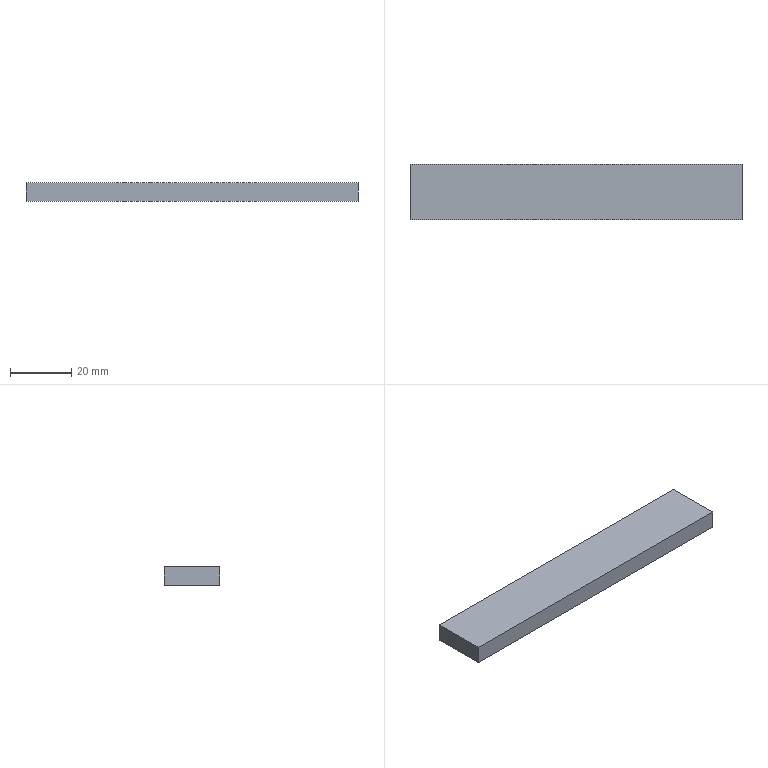Component | NX | TRANSFER_SURFACE_32 | 1 solid | 6 faces | box 108 x 18 x 6 mm | volume 11664 mm3 | plane 6
STEP:
#1=CARTESIAN_POINT('',(0.,0.,0.));
#2=DIRECTION('',(0.,0.,1.));
#3=DIRECTION('',(1.,0.,0.));
#4=AXIS2_PLACEMENT_3D('',#1,#2,#3);
#5=CARTESIAN_POINT('',(-115.,9.,12.));
#6=VERTEX_POINT('',#5);
#7=CARTESIAN_POINT('',(-115.,9.,6.));
#8=VERTEX_POINT('',#7);
#9=CARTESIAN_POINT('',(-115.,9.,12.));
#10=DIRECTION('',(0.,0.,-1.));
#11=VECTOR('',#10,1.);
#12=LINE('',#9,#11);
#13=CARTESIAN_POINT('',(-7.,9.,12.));
#14=DIRECTION('',(0.,1.,0.));
#15=DIRECTION('',(0.,0.,-1.));
#16=AXIS2_PLACEMENT_3D('',#13,#14,#15);
#17=PLANE('',#16);
#18=CARTESIAN_POINT('',(0.,108.));
#19=DIRECTION('',(1.,0.));
#20=VECTOR('',#19,1.);
#21=LINE('',#18,#20);
#22=(GEOMETRIC_REPRESENTATION_CONTEXT(2)PARAMETRIC_REPRESENTATION_CONTEXT()REPRESENTATION_CONTEXT('',''));
#23=DEFINITIONAL_REPRESENTATION('',(#21),#22);
#24=PCURVE('',#17,#23);
#25=CARTESIAN_POINT('',(-115.,9.,6.));
#26=DIRECTION('',(1.,0.,0.));
#27=DIRECTION('',(0.,0.,-1.));
#28=AXIS2_PLACEMENT_3D('',#25,#26,#27);
#29=PLANE('',#28);
#30=CARTESIAN_POINT('',(-6.,0.));
#31=DIRECTION('',(1.,0.));
#32=VECTOR('',#31,1.);
#33=LINE('',#30,#32);
#34=(GEOMETRIC_REPRESENTATION_CONTEXT(2)PARAMETRIC_REPRESENTATION_CONTEXT()REPRESENTATION_CONTEXT('',''));
#35=DEFINITIONAL_REPRESENTATION('',(#33),#34);
#36=PCURVE('',#29,#35);
#37=SURFACE_CURVE('',#12,(#24,#36),.PCURVE_S1.);
#38=EDGE_CURVE('',#6,#8,#37,.T.);
#39=ORIENTED_EDGE('',*,*,#38,.T.);
#40=CARTESIAN_POINT('',(-7.,9.,6.));
#41=VERTEX_POINT('',#40);
#42=CARTESIAN_POINT('',(-7.,9.,6.));
#43=DIRECTION('',(-1.,0.,0.));
#44=VECTOR('',#43,1.);
#45=LINE('',#42,#44);
#46=CARTESIAN_POINT('',(6.,0.));
#47=DIRECTION('',(0.,1.));
#48=VECTOR('',#47,1.);
#49=LINE('',#46,#48);
#50=(GEOMETRIC_REPRESENTATION_CONTEXT(2)PARAMETRIC_REPRESENTATION_CONTEXT()REPRESENTATION_CONTEXT('',''));
#51=DEFINITIONAL_REPRESENTATION('',(#49),#50);
#52=PCURVE('',#17,#51);
#53=CARTESIAN_POINT('',(-7.,9.,6.));
#54=DIRECTION('',(0.,0.,1.));
#55=DIRECTION('',(0.,1.,0.));
#56=AXIS2_PLACEMENT_3D('',#53,#54,#55);
#57=PLANE('',#56);
#58=CARTESIAN_POINT('',(0.,0.));
#59=DIRECTION('',(0.,1.));
#60=VECTOR('',#59,1.);
#61=LINE('',#58,#60);
#62=(GEOMETRIC_REPRESENTATION_CONTEXT(2)PARAMETRIC_REPRESENTATION_CONTEXT()REPRESENTATION_CONTEXT('',''));
#63=DEFINITIONAL_REPRESENTATION('',(#61),#62);
#64=PCURVE('',#57,#63);
#65=SURFACE_CURVE('',#45,(#52,#64),.PCURVE_S1.);
#66=EDGE_CURVE('',#41,#8,#65,.T.);
#67=ORIENTED_EDGE('',*,*,#66,.F.);
#68=CARTESIAN_POINT('',(-7.,9.,12.));
#69=VERTEX_POINT('',#68);
#70=CARTESIAN_POINT('',(-7.,9.,12.));
#71=DIRECTION('',(0.,0.,-1.));
#72=VECTOR('',#71,1.);
#73=LINE('',#70,#72);
#74=CARTESIAN_POINT('',(0.,0.));
#75=DIRECTION('',(1.,0.));
#76=VECTOR('',#75,1.);
#77=LINE('',#74,#76);
#78=(GEOMETRIC_REPRESENTATION_CONTEXT(2)PARAMETRIC_REPRESENTATION_CONTEXT()REPRESENTATION_CONTEXT('',''));
#79=DEFINITIONAL_REPRESENTATION('',(#77),#78);
#80=PCURVE('',#17,#79);
#81=CARTESIAN_POINT('',(-7.,9.,6.));
#82=DIRECTION('',(1.,0.,0.));
#83=DIRECTION('',(0.,0.,-1.));
#84=AXIS2_PLACEMENT_3D('',#81,#82,#83);
#85=PLANE('',#84);
#86=CARTESIAN_POINT('',(-6.,0.));
#87=DIRECTION('',(1.,0.));
#88=VECTOR('',#87,1.);
#89=LINE('',#86,#88);
#90=(GEOMETRIC_REPRESENTATION_CONTEXT(2)PARAMETRIC_REPRESENTATION_CONTEXT()REPRESENTATION_CONTEXT('',''));
#91=DEFINITIONAL_REPRESENTATION('',(#89),#90);
#92=PCURVE('',#85,#91);
#93=SURFACE_CURVE('',#73,(#80,#92),.PCURVE_S1.);
#94=EDGE_CURVE('',#69,#41,#93,.T.);
#95=ORIENTED_EDGE('',*,*,#94,.F.);
#96=CARTESIAN_POINT('',(-7.,9.,12.));
#97=DIRECTION('',(-1.,0.,0.));
#98=VECTOR('',#97,1.);
#99=LINE('',#96,#98);
#100=CARTESIAN_POINT('',(0.,0.));
#101=DIRECTION('',(0.,1.));
#102=VECTOR('',#101,1.);
#103=LINE('',#100,#102);
#104=(GEOMETRIC_REPRESENTATION_CONTEXT(2)PARAMETRIC_REPRESENTATION_CONTEXT()REPRESENTATION_CONTEXT('',''));
#105=DEFINITIONAL_REPRESENTATION('',(#103),#104);
#106=PCURVE('',#17,#105);
#107=CARTESIAN_POINT('',(-7.,27.,12.));
#108=DIRECTION('',(0.,0.,-1.));
#109=DIRECTION('',(0.,-1.,-0.));
#110=AXIS2_PLACEMENT_3D('',#107,#108,#109);
#111=PLANE('',#110);
#112=CARTESIAN_POINT('',(18.,0.));
#113=DIRECTION('',(0.,1.));
#114=VECTOR('',#113,1.);
#115=LINE('',#112,#114);
#116=(GEOMETRIC_REPRESENTATION_CONTEXT(2)PARAMETRIC_REPRESENTATION_CONTEXT()REPRESENTATION_CONTEXT('',''));
#117=DEFINITIONAL_REPRESENTATION('',(#115),#116);
#118=PCURVE('',#111,#117);
#119=SURFACE_CURVE('',#99,(#106,#118),.PCURVE_S1.);
#120=EDGE_CURVE('',#69,#6,#119,.T.);
#121=ORIENTED_EDGE('',*,*,#120,.T.);
#122=EDGE_LOOP('',(#39,#67,#95,#121));
#123=FACE_BOUND('',#122,.T.);
#124=ADVANCED_FACE('',(#123),#17,.F.);
#125=CARTESIAN_POINT('',(-115.,27.,6.));
#126=VERTEX_POINT('',#125);
#127=CARTESIAN_POINT('',(-115.,9.,6.));
#128=DIRECTION('',(0.,1.,0.));
#129=VECTOR('',#128,1.);
#130=LINE('',#127,#129);
#131=CARTESIAN_POINT('',(0.,108.));
#132=DIRECTION('',(1.,0.));
#133=VECTOR('',#132,1.);
#134=LINE('',#131,#133);
#135=(GEOMETRIC_REPRESENTATION_CONTEXT(2)PARAMETRIC_REPRESENTATION_CONTEXT()REPRESENTATION_CONTEXT('',''));
#136=DEFINITIONAL_REPRESENTATION('',(#134),#135);
#137=PCURVE('',#57,#136);
#138=CARTESIAN_POINT('',(0.,0.));
#139=DIRECTION('',(0.,1.));
#140=VECTOR('',#139,1.);
#141=LINE('',#138,#140);
#142=(GEOMETRIC_REPRESENTATION_CONTEXT(2)PARAMETRIC_REPRESENTATION_CONTEXT()REPRESENTATION_CONTEXT('',''));
#143=DEFINITIONAL_REPRESENTATION('',(#141),#142);
#144=PCURVE('',#29,#143);
#145=SURFACE_CURVE('',#130,(#137,#144),.PCURVE_S1.);
#146=EDGE_CURVE('',#8,#126,#145,.T.);
#147=ORIENTED_EDGE('',*,*,#146,.T.);
#148=CARTESIAN_POINT('',(-7.,27.,6.));
#149=VERTEX_POINT('',#148);
#150=CARTESIAN_POINT('',(-7.,27.,6.));
#151=DIRECTION('',(-1.,0.,0.));
#152=VECTOR('',#151,1.);
#153=LINE('',#150,#152);
#154=CARTESIAN_POINT('',(18.,0.));
#155=DIRECTION('',(0.,1.));
#156=VECTOR('',#155,1.);
#157=LINE('',#154,#156);
#158=(GEOMETRIC_REPRESENTATION_CONTEXT(2)PARAMETRIC_REPRESENTATION_CONTEXT()REPRESENTATION_CONTEXT('',''));
#159=DEFINITIONAL_REPRESENTATION('',(#157),#158);
#160=PCURVE('',#57,#159);
#161=CARTESIAN_POINT('',(-7.,27.,6.));
#162=DIRECTION('',(0.,-1.,-0.));
#163=DIRECTION('',(0.,-0.,1.));
#164=AXIS2_PLACEMENT_3D('',#161,#162,#163);
#165=PLANE('',#164);
#166=CARTESIAN_POINT('',(0.,0.));
#167=DIRECTION('',(0.,1.));
#168=VECTOR('',#167,1.);
#169=LINE('',#166,#168);
#170=(GEOMETRIC_REPRESENTATION_CONTEXT(2)PARAMETRIC_REPRESENTATION_CONTEXT()REPRESENTATION_CONTEXT('',''));
#171=DEFINITIONAL_REPRESENTATION('',(#169),#170);
#172=PCURVE('',#165,#171);
#173=SURFACE_CURVE('',#153,(#160,#172),.PCURVE_S1.);
#174=EDGE_CURVE('',#149,#126,#173,.T.);
#175=ORIENTED_EDGE('',*,*,#174,.F.);
#176=CARTESIAN_POINT('',(-7.,9.,6.));
#177=DIRECTION('',(0.,1.,0.));
#178=VECTOR('',#177,1.);
#179=LINE('',#176,#178);
#180=CARTESIAN_POINT('',(0.,0.));
#181=DIRECTION('',(1.,0.));
#182=VECTOR('',#181,1.);
#183=LINE('',#180,#182);
#184=(GEOMETRIC_REPRESENTATION_CONTEXT(2)PARAMETRIC_REPRESENTATION_CONTEXT()REPRESENTATION_CONTEXT('',''));
#185=DEFINITIONAL_REPRESENTATION('',(#183),#184);
#186=PCURVE('',#57,#185);
#187=CARTESIAN_POINT('',(0.,0.));
#188=DIRECTION('',(0.,1.));
#189=VECTOR('',#188,1.);
#190=LINE('',#187,#189);
#191=(GEOMETRIC_REPRESENTATION_CONTEXT(2)PARAMETRIC_REPRESENTATION_CONTEXT()REPRESENTATION_CONTEXT('',''));
#192=DEFINITIONAL_REPRESENTATION('',(#190),#191);
#193=PCURVE('',#85,#192);
#194=SURFACE_CURVE('',#179,(#186,#193),.PCURVE_S1.);
#195=EDGE_CURVE('',#41,#149,#194,.T.);
#196=ORIENTED_EDGE('',*,*,#195,.F.);
#197=ORIENTED_EDGE('',*,*,#66,.T.);
#198=EDGE_LOOP('',(#147,#175,#196,#197));
#199=FACE_BOUND('',#198,.T.);
#200=ADVANCED_FACE('',(#199),#57,.F.);
#201=CARTESIAN_POINT('',(-115.,27.,12.));
#202=VERTEX_POINT('',#201);
#203=CARTESIAN_POINT('',(-115.,27.,6.));
#204=DIRECTION('',(0.,-0.,1.));
#205=VECTOR('',#204,1.);
#206=LINE('',#203,#205);
#207=CARTESIAN_POINT('',(0.,108.));
#208=DIRECTION('',(1.,0.));
#209=VECTOR('',#208,1.);
#210=LINE('',#207,#209);
#211=(GEOMETRIC_REPRESENTATION_CONTEXT(2)PARAMETRIC_REPRESENTATION_CONTEXT()REPRESENTATION_CONTEXT('',''));
#212=DEFINITIONAL_REPRESENTATION('',(#210),#211);
#213=PCURVE('',#165,#212);
#214=CARTESIAN_POINT('',(0.,18.));
#215=DIRECTION('',(-1.,-0.));
#216=VECTOR('',#215,1.);
#217=LINE('',#214,#216);
#218=(GEOMETRIC_REPRESENTATION_CONTEXT(2)PARAMETRIC_REPRESENTATION_CONTEXT()REPRESENTATION_CONTEXT('',''));
#219=DEFINITIONAL_REPRESENTATION('',(#217),#218);
#220=PCURVE('',#29,#219);
#221=SURFACE_CURVE('',#206,(#213,#220),.PCURVE_S1.);
#222=EDGE_CURVE('',#126,#202,#221,.T.);
#223=ORIENTED_EDGE('',*,*,#222,.T.);
#224=CARTESIAN_POINT('',(-7.,27.,12.));
#225=VERTEX_POINT('',#224);
#226=CARTESIAN_POINT('',(-7.,27.,12.));
#227=DIRECTION('',(-1.,0.,0.));
#228=VECTOR('',#227,1.);
#229=LINE('',#226,#228);
#230=CARTESIAN_POINT('',(6.,0.));
#231=DIRECTION('',(0.,1.));
#232=VECTOR('',#231,1.);
#233=LINE('',#230,#232);
#234=(GEOMETRIC_REPRESENTATION_CONTEXT(2)PARAMETRIC_REPRESENTATION_CONTEXT()REPRESENTATION_CONTEXT('',''));
#235=DEFINITIONAL_REPRESENTATION('',(#233),#234);
#236=PCURVE('',#165,#235);
#237=CARTESIAN_POINT('',(0.,0.));
#238=DIRECTION('',(0.,1.));
#239=VECTOR('',#238,1.);
#240=LINE('',#237,#239);
#241=(GEOMETRIC_REPRESENTATION_CONTEXT(2)PARAMETRIC_REPRESENTATION_CONTEXT()REPRESENTATION_CONTEXT('',''));
#242=DEFINITIONAL_REPRESENTATION('',(#240),#241);
#243=PCURVE('',#111,#242);
#244=SURFACE_CURVE('',#229,(#236,#243),.PCURVE_S1.);
#245=EDGE_CURVE('',#225,#202,#244,.T.);
#246=ORIENTED_EDGE('',*,*,#245,.F.);
#247=CARTESIAN_POINT('',(-7.,27.,6.));
#248=DIRECTION('',(0.,-0.,1.));
#249=VECTOR('',#248,1.);
#250=LINE('',#247,#249);
#251=CARTESIAN_POINT('',(0.,0.));
#252=DIRECTION('',(1.,0.));
#253=VECTOR('',#252,1.);
#254=LINE('',#251,#253);
#255=(GEOMETRIC_REPRESENTATION_CONTEXT(2)PARAMETRIC_REPRESENTATION_CONTEXT()REPRESENTATION_CONTEXT('',''));
#256=DEFINITIONAL_REPRESENTATION('',(#254),#255);
#257=PCURVE('',#165,#256);
#258=CARTESIAN_POINT('',(0.,18.));
#259=DIRECTION('',(-1.,-0.));
#260=VECTOR('',#259,1.);
#261=LINE('',#258,#260);
#262=(GEOMETRIC_REPRESENTATION_CONTEXT(2)PARAMETRIC_REPRESENTATION_CONTEXT()REPRESENTATION_CONTEXT('',''));
#263=DEFINITIONAL_REPRESENTATION('',(#261),#262);
#264=PCURVE('',#85,#263);
#265=SURFACE_CURVE('',#250,(#257,#264),.PCURVE_S1.);
#266=EDGE_CURVE('',#149,#225,#265,.T.);
#267=ORIENTED_EDGE('',*,*,#266,.F.);
#268=ORIENTED_EDGE('',*,*,#174,.T.);
#269=EDGE_LOOP('',(#223,#246,#267,#268));
#270=FACE_BOUND('',#269,.T.);
#271=ADVANCED_FACE('',(#270),#165,.F.);
#272=CARTESIAN_POINT('',(-115.,27.,12.));
#273=DIRECTION('',(0.,-1.,-0.));
#274=VECTOR('',#273,1.);
#275=LINE('',#272,#274);
#276=CARTESIAN_POINT('',(0.,108.));
#277=DIRECTION('',(1.,0.));
#278=VECTOR('',#277,1.);
#279=LINE('',#276,#278);
#280=(GEOMETRIC_REPRESENTATION_CONTEXT(2)PARAMETRIC_REPRESENTATION_CONTEXT()REPRESENTATION_CONTEXT('',''));
#281=DEFINITIONAL_REPRESENTATION('',(#279),#280);
#282=PCURVE('',#111,#281);
#283=CARTESIAN_POINT('',(-6.,18.));
#284=DIRECTION('',(0.,-1.));
#285=VECTOR('',#284,1.);
#286=LINE('',#283,#285);
#287=(GEOMETRIC_REPRESENTATION_CONTEXT(2)PARAMETRIC_REPRESENTATION_CONTEXT()REPRESENTATION_CONTEXT('',''));
#288=DEFINITIONAL_REPRESENTATION('',(#286),#287);
#289=PCURVE('',#29,#288);
#290=SURFACE_CURVE('',#275,(#282,#289),.PCURVE_S1.);
#291=EDGE_CURVE('',#202,#6,#290,.T.);
#292=ORIENTED_EDGE('',*,*,#291,.T.);
#293=ORIENTED_EDGE('',*,*,#120,.F.);
#294=CARTESIAN_POINT('',(-7.,27.,12.));
#295=DIRECTION('',(0.,-1.,-0.));
#296=VECTOR('',#295,1.);
#297=LINE('',#294,#296);
#298=CARTESIAN_POINT('',(0.,0.));
#299=DIRECTION('',(1.,0.));
#300=VECTOR('',#299,1.);
#301=LINE('',#298,#300);
#302=(GEOMETRIC_REPRESENTATION_CONTEXT(2)PARAMETRIC_REPRESENTATION_CONTEXT()REPRESENTATION_CONTEXT('',''));
#303=DEFINITIONAL_REPRESENTATION('',(#301),#302);
#304=PCURVE('',#111,#303);
#305=CARTESIAN_POINT('',(-6.,18.));
#306=DIRECTION('',(0.,-1.));
#307=VECTOR('',#306,1.);
#308=LINE('',#305,#307);
#309=(GEOMETRIC_REPRESENTATION_CONTEXT(2)PARAMETRIC_REPRESENTATION_CONTEXT()REPRESENTATION_CONTEXT('',''));
#310=DEFINITIONAL_REPRESENTATION('',(#308),#309);
#311=PCURVE('',#85,#310);
#312=SURFACE_CURVE('',#297,(#304,#311),.PCURVE_S1.);
#313=EDGE_CURVE('',#225,#69,#312,.T.);
#314=ORIENTED_EDGE('',*,*,#313,.F.);
#315=ORIENTED_EDGE('',*,*,#245,.T.);
#316=EDGE_LOOP('',(#292,#293,#314,#315));
#317=FACE_BOUND('',#316,.T.);
#318=ADVANCED_FACE('',(#317),#111,.F.);
#319=ORIENTED_EDGE('',*,*,#94,.T.);
#320=ORIENTED_EDGE('',*,*,#195,.T.);
#321=ORIENTED_EDGE('',*,*,#266,.T.);
#322=ORIENTED_EDGE('',*,*,#313,.T.);
#323=EDGE_LOOP('',(#319,#320,#321,#322));
#324=FACE_BOUND('',#323,.T.);
#325=ADVANCED_FACE('',(#324),#85,.T.);
#326=ORIENTED_EDGE('',*,*,#38,.F.);
#327=ORIENTED_EDGE('',*,*,#291,.F.);
#328=ORIENTED_EDGE('',*,*,#222,.F.);
#329=ORIENTED_EDGE('',*,*,#146,.F.);
#330=EDGE_LOOP('',(#326,#327,#328,#329));
#331=FACE_BOUND('',#330,.T.);
#332=ADVANCED_FACE('',(#331),#29,.F.);
#333=CLOSED_SHELL('',(#124,#200,#271,#318,#325,#332));
#334=MANIFOLD_SOLID_BREP('',#333);
#335=(LENGTH_UNIT()NAMED_UNIT(*)SI_UNIT(.MILLI.,.METRE.));
#336=UNCERTAINTY_MEASURE_WITH_UNIT(LENGTH_MEASURE(0.0000001),#335,'','');
#337=(NAMED_UNIT(*)PLANE_ANGLE_UNIT()SI_UNIT($,.RADIAN.));
#338=(NAMED_UNIT(*)SI_UNIT($,.STERADIAN.)SOLID_ANGLE_UNIT());
#339=(GEOMETRIC_REPRESENTATION_CONTEXT(3)GLOBAL_UNCERTAINTY_ASSIGNED_CONTEXT((#336))GLOBAL_UNIT_ASSIGNED_CONTEXT((#335,#337,#338))REPRESENTATION_CONTEXT('',''));
#340=ADVANCED_BREP_SHAPE_REPRESENTATION('',(#4,#334),#339);